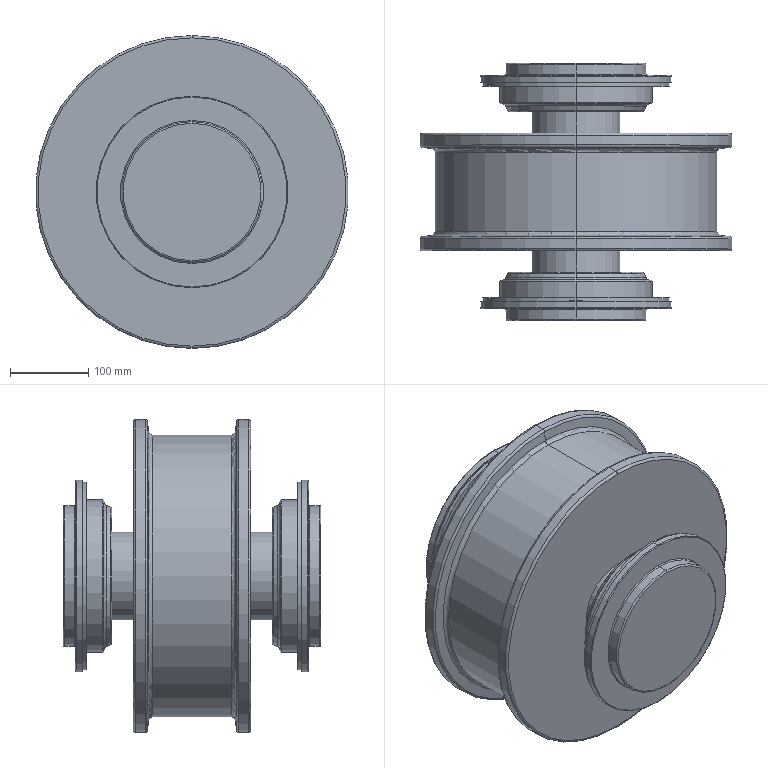Component | SolidWorks | WheelFrom-3 | 1 solid | 88 faces | box 400 x 329 x 400 mm | volume 20648982 mm3 | torus 36 | cylinder 26 | plane 14 | cone 12 | commonest cylinder face diameters 180 x4 245 x4 240 x4 195 x4 112 x4 400 x4 360 x2 | material Plain Carbon Steel
build123d program:
from build123d import *

# Parameters (mm, degrees)
CUT_EXTRUDE1_DEPTH      = 3
CUT_EXTRUDE1_DEPTH_BACK = 3
CUT_EXTRUDE1_START      = 29
CUT_EXTRUDE2_DEPTH      = 624.362
CUT_EXTRUDE2_DEPTH_BACK = 624.362
SKETCH4_W               = 243.271
SKETCH4_H               = 102.964


with BuildPart() as part:
    # Sketch2 → Revolve1 (revolve)
    with BuildSketch(Plane.XY):
        with BuildLine():
            Line((0, 0), (0, 29))
            Line((0, 29), (-3.5, 30))
            Line((-3.5, 30), (-208, 30))
            Line((-208, 30), (-208, 35.5))
            Line((-208, 35.5), (-210, 37.5))
            Line((-210, 37.5), (-226.5, 37.5))
            Line((-226.5, 37.5), (-226.5, 88))
            ThreePointArc((-226.5, 88), (-227.086, 89.414), (-228.5, 90))
            Line((-228.5, 90), (-240.5, 90))
            ThreePointArc((-240.5, 90), (-241.561, 90.439), (-242, 91.5))
            Line((-242, 91.5), (-242, 121.5))
            ThreePointArc((-242, 121.5), (-242.293, 122.207), (-243, 122.5))
            Line((-243, 122.5), (-251, 122.5))
            Line((-251, 122.5), (-251, 120.5))
            ThreePointArc((-251, 120.5), (-251.146, 120.146), (-251.5, 120))
            Line((-251.5, 120), (-256, 120))
            Line((-256, 120), (-256, 97.5))
            Line((-256, 97.5), (-277, 97.5))
            Line((-277, 97.5), (-278.5, 96.5))
            Line((-278.5, 96.5), (-278.5, 94.474))
            ThreePointArc((-278.5, 94.474), (-279.237, 91.977), (-281.212, 90.279))
            Line((-281.212, 90.279), (-287.049, 87.653))
            ThreePointArc((-287.049, 87.653), (-288.106, 86.745), (-288.5, 85.409))
            Line((-288.5, 85.409), (-288.5, 56))
            Line((-288.5, 56), (-316, 56))
            Line((-316, 56), (-316, 197))
            ThreePointArc((-316, 197), (-316.879, 199.121), (-319, 200))
            Line((-319, 200), (-331.199, 200))
            ThreePointArc((-331.199, 200), (-333.206, 199.229), (-334.182, 197.313))
            Line((-334.182, 197.313), (-335.53, 184.478))
            ThreePointArc((-335.53, 184.478), (-337.157, 181.284), (-340.502, 180))
            Line((-340.502, 180), (-441.498, 180))
            ThreePointArc((-441.498, 180), (-444.843, 181.284), (-446.47, 184.478))
            Line((-446.47, 184.478), (-447.818, 197.313))
            ThreePointArc((-447.818, 197.313), (-448.794, 199.229), (-450.801, 200))
            Line((-450.801, 200), (-463, 200))
            ThreePointArc((-463, 200), (-465.121, 199.121), (-466, 197))
            Line((-466, 197), (-466, 56))
            Line((-466, 56), (-493.5, 56))
            Line((-493.5, 56), (-493.5, 85.409))
            ThreePointArc((-493.5, 85.409), (-493.894, 86.745), (-494.951, 87.653))
            Line((-494.951, 87.653), (-500.788, 90.279))
            ThreePointArc((-500.788, 90.279), (-502.763, 91.977), (-503.5, 94.474))
            Line((-503.5, 94.474), (-503.5, 96.5))
            Line((-503.5, 96.5), (-505, 97.5))
            Line((-505, 97.5), (-526, 97.5))
            Line((-526, 97.5), (-526, 120))
            Line((-526, 120), (-530.5, 120))
            ThreePointArc((-530.5, 120), (-530.854, 120.146), (-531, 120.5))
            Line((-531, 120.5), (-531, 122.5))
            Line((-531, 122.5), (-539, 122.5))
            ThreePointArc((-539, 122.5), (-539.707, 122.207), (-540, 121.5))
            Line((-540, 121.5), (-540, 91.5))
            ThreePointArc((-540, 91.5), (-540.439, 90.439), (-541.5, 90))
            Line((-541.5, 90), (-553.5, 90))
            ThreePointArc((-553.5, 90), (-554.914, 89.414), (-555.5, 88))
            Line((-555.5, 88), (-555.5, 0))
            Line((-555.5, 0), (0, 0))
        make_face()
    revolve(axis=Axis((0, 0, 0), (-1, 0, 0)))

    # Sketch3 → Cut-Extrude1 (cut, two sides: drawn at the far end of the back side and taken through both)
    with BuildSketch(Plane.XY.offset(CUT_EXTRUDE1_START - CUT_EXTRUDE1_DEPTH_BACK)):
        with BuildLine():
            Line((-186, 9), (-24, 9))
            ThreePointArc((-24, 9), (-15, 0), (-24, -9))
            Line((-24, -9), (-186, -9))
            ThreePointArc((-186, -9), (-195, 0), (-186, 9))
        make_face()
    extrude(amount=CUT_EXTRUDE1_DEPTH + CUT_EXTRUDE1_DEPTH_BACK, mode=Mode.SUBTRACT)

    # Sketch4 → Cut-Extrude2 (cut, two sides: drawn at the far end of the back side and taken through both)
    with BuildSketch(Plane.XY.offset(-CUT_EXTRUDE2_DEPTH_BACK)):
        with Locations((-104.864, 8.078)):
            Rectangle(SKETCH4_W, SKETCH4_H)
    extrude(amount=CUT_EXTRUDE2_DEPTH + CUT_EXTRUDE2_DEPTH_BACK, mode=Mode.SUBTRACT)


solid = part.part

# Placed as in the assembly
solid = solid.moved(Location((550.579, 1647.349, 2003.088), (0, 0, 90)))